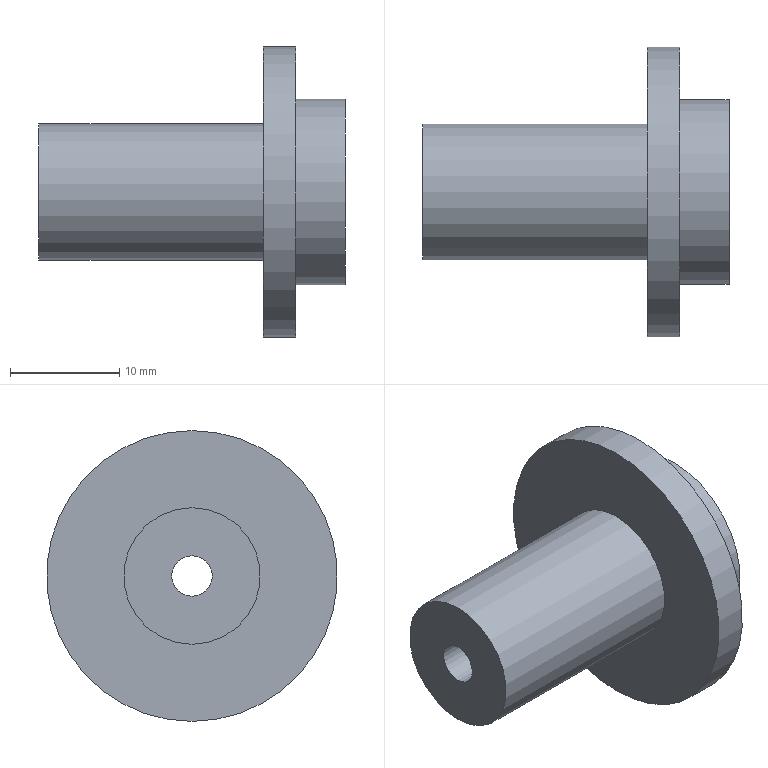Component | NX | FLOW_SEAT | 1 solid | 8 faces | box 28 x 26.6 x 26.6 mm | volume 4903 mm3 | cylinder 4 | plane 4 | commonest cylinder face diameters 12.5 x1 26.6 x1 17 x1 3.7 x1
STEP:
#1=CARTESIAN_POINT('',(0.,0.,0.));
#2=DIRECTION('',(0.,0.,1.));
#3=DIRECTION('',(1.,0.,0.));
#4=AXIS2_PLACEMENT_3D('',#1,#2,#3);
#5=CARTESIAN_POINT('',(-8.,-0.,13.75));
#6=VERTEX_POINT('',#5);
#7=CARTESIAN_POINT('',(-8.,-0.,20.));
#8=DIRECTION('',(1.,0.,0.));
#9=DIRECTION('',(0.,0.,-1.));
#10=AXIS2_PLACEMENT_3D('',#7,#8,#9);
#11=CIRCLE('',#10,6.25);
#12=CARTESIAN_POINT('',(-8.,-0.,20.));
#13=DIRECTION('',(-1.,0.,0.));
#14=DIRECTION('',(0.,0.,1.));
#15=AXIS2_PLACEMENT_3D('',#12,#13,#14);
#16=CYLINDRICAL_SURFACE('',#15,6.25);
#17=CARTESIAN_POINT('',(9.425,0.));
#18=DIRECTION('',(-1.,0.));
#19=VECTOR('',#18,1.);
#20=LINE('',#17,#19);
#21=(GEOMETRIC_REPRESENTATION_CONTEXT(2)PARAMETRIC_REPRESENTATION_CONTEXT()REPRESENTATION_CONTEXT('',''));
#22=DEFINITIONAL_REPRESENTATION('',(#20),#21);
#23=PCURVE('',#16,#22);
#24=CARTESIAN_POINT('',(-8.,-0.,20.));
#25=DIRECTION('',(1.,0.,0.));
#26=DIRECTION('',(0.,0.,-1.));
#27=AXIS2_PLACEMENT_3D('',#24,#25,#26);
#28=PLANE('',#27);
#29=CARTESIAN_POINT('',(0.,0.));
#30=DIRECTION('',(1.,0.));
#31=AXIS2_PLACEMENT_2D('',#29,#30);
#32=CIRCLE('',#31,6.25);
#33=(GEOMETRIC_REPRESENTATION_CONTEXT(2)PARAMETRIC_REPRESENTATION_CONTEXT()REPRESENTATION_CONTEXT('',''));
#34=DEFINITIONAL_REPRESENTATION('',(#32),#33);
#35=PCURVE('',#28,#34);
#36=SURFACE_CURVE('',#11,(#23,#35),.PCURVE_S1.);
#37=EDGE_CURVE('',#6,#6,#36,.T.);
#38=ORIENTED_EDGE('',*,*,#37,.F.);
#39=CARTESIAN_POINT('',(-28.5,-0.,13.75));
#40=VERTEX_POINT('',#39);
#41=CARTESIAN_POINT('',(-8.,-0.,13.75));
#42=CARTESIAN_POINT('',(-28.5,-0.,13.75));
#43=B_SPLINE_CURVE_WITH_KNOTS('',1,(#41,#42),.UNSPECIFIED.,.F.,.F.,(2,2),(0.,20.5),.PIECEWISE_BEZIER_KNOTS.);
#44=CARTESIAN_POINT('',(9.425,0.));
#45=DIRECTION('',(0.,1.));
#46=VECTOR('',#45,1.);
#47=LINE('',#44,#46);
#48=(GEOMETRIC_REPRESENTATION_CONTEXT(2)PARAMETRIC_REPRESENTATION_CONTEXT()REPRESENTATION_CONTEXT('',''));
#49=DEFINITIONAL_REPRESENTATION('',(#47),#48);
#50=PCURVE('',#16,#49);
#51=CARTESIAN_POINT('',(3.142,0.));
#52=DIRECTION('',(0.,1.));
#53=VECTOR('',#52,1.);
#54=LINE('',#51,#53);
#55=(GEOMETRIC_REPRESENTATION_CONTEXT(2)PARAMETRIC_REPRESENTATION_CONTEXT()REPRESENTATION_CONTEXT('',''));
#56=DEFINITIONAL_REPRESENTATION('',(#54),#55);
#57=PCURVE('',#16,#56);
#58=SEAM_CURVE('',#43,(#50,#57),.PCURVE_S1.);
#59=EDGE_CURVE('',#6,#40,#58,.T.);
#60=ORIENTED_EDGE('',*,*,#59,.T.);
#61=CARTESIAN_POINT('',(-28.5,-0.,20.));
#62=DIRECTION('',(1.,0.,0.));
#63=DIRECTION('',(0.,0.,-1.));
#64=AXIS2_PLACEMENT_3D('',#61,#62,#63);
#65=CIRCLE('',#64,6.25);
#66=CARTESIAN_POINT('',(9.425,20.5));
#67=DIRECTION('',(-1.,0.));
#68=VECTOR('',#67,1.);
#69=LINE('',#66,#68);
#70=(GEOMETRIC_REPRESENTATION_CONTEXT(2)PARAMETRIC_REPRESENTATION_CONTEXT()REPRESENTATION_CONTEXT('',''));
#71=DEFINITIONAL_REPRESENTATION('',(#69),#70);
#72=PCURVE('',#16,#71);
#73=CARTESIAN_POINT('',(-28.5,-0.,20.));
#74=DIRECTION('',(1.,0.,0.));
#75=DIRECTION('',(0.,0.,-1.));
#76=AXIS2_PLACEMENT_3D('',#73,#74,#75);
#77=PLANE('',#76);
#78=CARTESIAN_POINT('',(0.,0.));
#79=DIRECTION('',(1.,0.));
#80=AXIS2_PLACEMENT_2D('',#78,#79);
#81=CIRCLE('',#80,6.25);
#82=(GEOMETRIC_REPRESENTATION_CONTEXT(2)PARAMETRIC_REPRESENTATION_CONTEXT()REPRESENTATION_CONTEXT('',''));
#83=DEFINITIONAL_REPRESENTATION('',(#81),#82);
#84=PCURVE('',#77,#83);
#85=SURFACE_CURVE('',#65,(#72,#84),.PCURVE_S1.);
#86=EDGE_CURVE('',#40,#40,#85,.T.);
#87=ORIENTED_EDGE('',*,*,#86,.T.);
#88=ORIENTED_EDGE('',*,*,#59,.F.);
#89=EDGE_LOOP('',(#38,#60,#87,#88));
#90=FACE_BOUND('',#89,.T.);
#91=ADVANCED_FACE('',(#90),#16,.T.);
#92=CARTESIAN_POINT('',(-28.5,-0.,18.15));
#93=VERTEX_POINT('',#92);
#94=CARTESIAN_POINT('',(-28.5,-0.,21.85));
#95=VERTEX_POINT('',#94);
#96=CARTESIAN_POINT('',(-28.5,-0.,20.));
#97=DIRECTION('',(1.,0.,0.));
#98=DIRECTION('',(0.,0.,-1.));
#99=AXIS2_PLACEMENT_3D('',#96,#97,#98);
#100=CIRCLE('',#99,1.85);
#101=CARTESIAN_POINT('',(0.,0.));
#102=DIRECTION('',(1.,0.));
#103=AXIS2_PLACEMENT_2D('',#101,#102);
#104=CIRCLE('',#103,1.85);
#105=(GEOMETRIC_REPRESENTATION_CONTEXT(2)PARAMETRIC_REPRESENTATION_CONTEXT()REPRESENTATION_CONTEXT('',''));
#106=DEFINITIONAL_REPRESENTATION('',(#104),#105);
#107=PCURVE('',#77,#106);
#108=CARTESIAN_POINT('',(-0.5,-0.,20.));
#109=DIRECTION('',(-1.,0.,0.));
#110=DIRECTION('',(0.,0.,1.));
#111=AXIS2_PLACEMENT_3D('',#108,#109,#110);
#112=CYLINDRICAL_SURFACE('',#111,1.85);
#113=CARTESIAN_POINT('',(3.142,28.));
#114=DIRECTION('',(-1.,0.));
#115=VECTOR('',#114,1.);
#116=LINE('',#113,#115);
#117=(GEOMETRIC_REPRESENTATION_CONTEXT(2)PARAMETRIC_REPRESENTATION_CONTEXT()REPRESENTATION_CONTEXT('',''));
#118=DEFINITIONAL_REPRESENTATION('',(#116),#117);
#119=PCURVE('',#112,#118);
#120=SURFACE_CURVE('',#100,(#107,#119),.PCURVE_S1.);
#121=EDGE_CURVE('',#93,#95,#120,.T.);
#122=ORIENTED_EDGE('',*,*,#121,.T.);
#123=CARTESIAN_POINT('',(-28.5,-0.,20.));
#124=DIRECTION('',(1.,0.,0.));
#125=DIRECTION('',(0.,0.,-1.));
#126=AXIS2_PLACEMENT_3D('',#123,#124,#125);
#127=CIRCLE('',#126,1.85);
#128=CARTESIAN_POINT('',(0.,0.));
#129=DIRECTION('',(1.,0.));
#130=AXIS2_PLACEMENT_2D('',#128,#129);
#131=CIRCLE('',#130,1.85);
#132=(GEOMETRIC_REPRESENTATION_CONTEXT(2)PARAMETRIC_REPRESENTATION_CONTEXT()REPRESENTATION_CONTEXT('',''));
#133=DEFINITIONAL_REPRESENTATION('',(#131),#132);
#134=PCURVE('',#77,#133);
#135=CARTESIAN_POINT('',(9.425,28.));
#136=DIRECTION('',(-1.,0.));
#137=VECTOR('',#136,1.);
#138=LINE('',#135,#137);
#139=(GEOMETRIC_REPRESENTATION_CONTEXT(2)PARAMETRIC_REPRESENTATION_CONTEXT()REPRESENTATION_CONTEXT('',''));
#140=DEFINITIONAL_REPRESENTATION('',(#138),#139);
#141=PCURVE('',#112,#140);
#142=SURFACE_CURVE('',#127,(#134,#141),.PCURVE_S1.);
#143=EDGE_CURVE('',#95,#93,#142,.T.);
#144=ORIENTED_EDGE('',*,*,#143,.T.);
#145=EDGE_LOOP('',(#122,#144));
#146=FACE_BOUND('',#145,.T.);
#147=ORIENTED_EDGE('',*,*,#86,.F.);
#148=EDGE_LOOP('',(#147));
#149=FACE_BOUND('',#148,.T.);
#150=ADVANCED_FACE('',(#146,#149),#77,.F.);
#151=CARTESIAN_POINT('',(-5.,-0.,6.7));
#152=VERTEX_POINT('',#151);
#153=CARTESIAN_POINT('',(-5.,-0.,20.));
#154=DIRECTION('',(1.,0.,0.));
#155=DIRECTION('',(0.,0.,-1.));
#156=AXIS2_PLACEMENT_3D('',#153,#154,#155);
#157=CIRCLE('',#156,13.3);
#158=CARTESIAN_POINT('',(-5.,-0.,20.));
#159=DIRECTION('',(-1.,0.,0.));
#160=DIRECTION('',(0.,0.,1.));
#161=AXIS2_PLACEMENT_3D('',#158,#159,#160);
#162=CYLINDRICAL_SURFACE('',#161,13.3);
#163=CARTESIAN_POINT('',(9.425,0.));
#164=DIRECTION('',(-1.,0.));
#165=VECTOR('',#164,1.);
#166=LINE('',#163,#165);
#167=(GEOMETRIC_REPRESENTATION_CONTEXT(2)PARAMETRIC_REPRESENTATION_CONTEXT()REPRESENTATION_CONTEXT('',''));
#168=DEFINITIONAL_REPRESENTATION('',(#166),#167);
#169=PCURVE('',#162,#168);
#170=CARTESIAN_POINT('',(-5.,-0.,20.));
#171=DIRECTION('',(1.,0.,0.));
#172=DIRECTION('',(0.,0.,-1.));
#173=AXIS2_PLACEMENT_3D('',#170,#171,#172);
#174=PLANE('',#173);
#175=CARTESIAN_POINT('',(0.,0.));
#176=DIRECTION('',(1.,0.));
#177=AXIS2_PLACEMENT_2D('',#175,#176);
#178=CIRCLE('',#177,13.3);
#179=(GEOMETRIC_REPRESENTATION_CONTEXT(2)PARAMETRIC_REPRESENTATION_CONTEXT()REPRESENTATION_CONTEXT('',''));
#180=DEFINITIONAL_REPRESENTATION('',(#178),#179);
#181=PCURVE('',#174,#180);
#182=SURFACE_CURVE('',#157,(#169,#181),.PCURVE_S1.);
#183=EDGE_CURVE('',#152,#152,#182,.T.);
#184=ORIENTED_EDGE('',*,*,#183,.F.);
#185=CARTESIAN_POINT('',(-8.,-0.,6.7));
#186=VERTEX_POINT('',#185);
#187=CARTESIAN_POINT('',(-5.,-0.,6.7));
#188=CARTESIAN_POINT('',(-8.,-0.,6.7));
#189=B_SPLINE_CURVE_WITH_KNOTS('',1,(#187,#188),.UNSPECIFIED.,.F.,.F.,(2,2),(0.,3.),.PIECEWISE_BEZIER_KNOTS.);
#190=CARTESIAN_POINT('',(9.425,0.));
#191=DIRECTION('',(0.,1.));
#192=VECTOR('',#191,1.);
#193=LINE('',#190,#192);
#194=(GEOMETRIC_REPRESENTATION_CONTEXT(2)PARAMETRIC_REPRESENTATION_CONTEXT()REPRESENTATION_CONTEXT('',''));
#195=DEFINITIONAL_REPRESENTATION('',(#193),#194);
#196=PCURVE('',#162,#195);
#197=CARTESIAN_POINT('',(3.142,0.));
#198=DIRECTION('',(0.,1.));
#199=VECTOR('',#198,1.);
#200=LINE('',#197,#199);
#201=(GEOMETRIC_REPRESENTATION_CONTEXT(2)PARAMETRIC_REPRESENTATION_CONTEXT()REPRESENTATION_CONTEXT('',''));
#202=DEFINITIONAL_REPRESENTATION('',(#200),#201);
#203=PCURVE('',#162,#202);
#204=SEAM_CURVE('',#189,(#196,#203),.PCURVE_S1.);
#205=EDGE_CURVE('',#152,#186,#204,.T.);
#206=ORIENTED_EDGE('',*,*,#205,.T.);
#207=CARTESIAN_POINT('',(-8.,-0.,20.));
#208=DIRECTION('',(1.,0.,0.));
#209=DIRECTION('',(0.,0.,-1.));
#210=AXIS2_PLACEMENT_3D('',#207,#208,#209);
#211=CIRCLE('',#210,13.3);
#212=CARTESIAN_POINT('',(9.425,3.));
#213=DIRECTION('',(-1.,0.));
#214=VECTOR('',#213,1.);
#215=LINE('',#212,#214);
#216=(GEOMETRIC_REPRESENTATION_CONTEXT(2)PARAMETRIC_REPRESENTATION_CONTEXT()REPRESENTATION_CONTEXT('',''));
#217=DEFINITIONAL_REPRESENTATION('',(#215),#216);
#218=PCURVE('',#162,#217);
#219=CARTESIAN_POINT('',(0.,0.));
#220=DIRECTION('',(1.,0.));
#221=AXIS2_PLACEMENT_2D('',#219,#220);
#222=CIRCLE('',#221,13.3);
#223=(GEOMETRIC_REPRESENTATION_CONTEXT(2)PARAMETRIC_REPRESENTATION_CONTEXT()REPRESENTATION_CONTEXT('',''));
#224=DEFINITIONAL_REPRESENTATION('',(#222),#223);
#225=PCURVE('',#28,#224);
#226=SURFACE_CURVE('',#211,(#218,#225),.PCURVE_S1.);
#227=EDGE_CURVE('',#186,#186,#226,.T.);
#228=ORIENTED_EDGE('',*,*,#227,.T.);
#229=ORIENTED_EDGE('',*,*,#205,.F.);
#230=EDGE_LOOP('',(#184,#206,#228,#229));
#231=FACE_BOUND('',#230,.T.);
#232=ADVANCED_FACE('',(#231),#162,.T.);
#233=CARTESIAN_POINT('',(-5.,-0.,11.5));
#234=VERTEX_POINT('',#233);
#235=CARTESIAN_POINT('',(-5.,-0.,20.));
#236=DIRECTION('',(1.,0.,0.));
#237=DIRECTION('',(0.,0.,-1.));
#238=AXIS2_PLACEMENT_3D('',#235,#236,#237);
#239=CIRCLE('',#238,8.5);
#240=CARTESIAN_POINT('',(0.,0.));
#241=DIRECTION('',(1.,0.));
#242=AXIS2_PLACEMENT_2D('',#240,#241);
#243=CIRCLE('',#242,8.5);
#244=(GEOMETRIC_REPRESENTATION_CONTEXT(2)PARAMETRIC_REPRESENTATION_CONTEXT()REPRESENTATION_CONTEXT('',''));
#245=DEFINITIONAL_REPRESENTATION('',(#243),#244);
#246=PCURVE('',#174,#245);
#247=CARTESIAN_POINT('',(-0.5,-0.,20.));
#248=DIRECTION('',(-1.,0.,0.));
#249=DIRECTION('',(0.,0.,1.));
#250=AXIS2_PLACEMENT_3D('',#247,#248,#249);
#251=CYLINDRICAL_SURFACE('',#250,8.5);
#252=CARTESIAN_POINT('',(9.425,4.5));
#253=DIRECTION('',(-1.,0.));
#254=VECTOR('',#253,1.);
#255=LINE('',#252,#254);
#256=(GEOMETRIC_REPRESENTATION_CONTEXT(2)PARAMETRIC_REPRESENTATION_CONTEXT()REPRESENTATION_CONTEXT('',''));
#257=DEFINITIONAL_REPRESENTATION('',(#255),#256);
#258=PCURVE('',#251,#257);
#259=SURFACE_CURVE('',#239,(#246,#258),.PCURVE_S1.);
#260=EDGE_CURVE('',#234,#234,#259,.T.);
#261=ORIENTED_EDGE('',*,*,#260,.F.);
#262=EDGE_LOOP('',(#261));
#263=FACE_BOUND('',#262,.T.);
#264=ORIENTED_EDGE('',*,*,#183,.T.);
#265=EDGE_LOOP('',(#264));
#266=FACE_BOUND('',#265,.T.);
#267=ADVANCED_FACE('',(#263,#266),#174,.T.);
#268=ORIENTED_EDGE('',*,*,#37,.T.);
#269=EDGE_LOOP('',(#268));
#270=FACE_BOUND('',#269,.T.);
#271=ORIENTED_EDGE('',*,*,#227,.F.);
#272=EDGE_LOOP('',(#271));
#273=FACE_BOUND('',#272,.T.);
#274=ADVANCED_FACE('',(#270,#273),#28,.F.);
#275=CARTESIAN_POINT('',(-0.5,-0.,11.5));
#276=VERTEX_POINT('',#275);
#277=CARTESIAN_POINT('',(-0.5,-0.,20.));
#278=DIRECTION('',(1.,0.,0.));
#279=DIRECTION('',(0.,0.,-1.));
#280=AXIS2_PLACEMENT_3D('',#277,#278,#279);
#281=CIRCLE('',#280,8.5);
#282=CARTESIAN_POINT('',(9.425,0.));
#283=DIRECTION('',(-1.,0.));
#284=VECTOR('',#283,1.);
#285=LINE('',#282,#284);
#286=(GEOMETRIC_REPRESENTATION_CONTEXT(2)PARAMETRIC_REPRESENTATION_CONTEXT()REPRESENTATION_CONTEXT('',''));
#287=DEFINITIONAL_REPRESENTATION('',(#285),#286);
#288=PCURVE('',#251,#287);
#289=CARTESIAN_POINT('',(-0.5,-0.,20.));
#290=DIRECTION('',(1.,0.,0.));
#291=DIRECTION('',(0.,0.,-1.));
#292=AXIS2_PLACEMENT_3D('',#289,#290,#291);
#293=PLANE('',#292);
#294=CARTESIAN_POINT('',(0.,0.));
#295=DIRECTION('',(1.,0.));
#296=AXIS2_PLACEMENT_2D('',#294,#295);
#297=CIRCLE('',#296,8.5);
#298=(GEOMETRIC_REPRESENTATION_CONTEXT(2)PARAMETRIC_REPRESENTATION_CONTEXT()REPRESENTATION_CONTEXT('',''));
#299=DEFINITIONAL_REPRESENTATION('',(#297),#298);
#300=PCURVE('',#293,#299);
#301=SURFACE_CURVE('',#281,(#288,#300),.PCURVE_S1.);
#302=EDGE_CURVE('',#276,#276,#301,.T.);
#303=ORIENTED_EDGE('',*,*,#302,.F.);
#304=CARTESIAN_POINT('',(-0.5,-0.,11.5));
#305=CARTESIAN_POINT('',(-5.,-0.,11.5));
#306=B_SPLINE_CURVE_WITH_KNOTS('',1,(#304,#305),.UNSPECIFIED.,.F.,.F.,(2,2),(0.,4.5),.PIECEWISE_BEZIER_KNOTS.);
#307=CARTESIAN_POINT('',(9.425,0.));
#308=DIRECTION('',(0.,1.));
#309=VECTOR('',#308,1.);
#310=LINE('',#307,#309);
#311=(GEOMETRIC_REPRESENTATION_CONTEXT(2)PARAMETRIC_REPRESENTATION_CONTEXT()REPRESENTATION_CONTEXT('',''));
#312=DEFINITIONAL_REPRESENTATION('',(#310),#311);
#313=PCURVE('',#251,#312);
#314=CARTESIAN_POINT('',(3.142,0.));
#315=DIRECTION('',(0.,1.));
#316=VECTOR('',#315,1.);
#317=LINE('',#314,#316);
#318=(GEOMETRIC_REPRESENTATION_CONTEXT(2)PARAMETRIC_REPRESENTATION_CONTEXT()REPRESENTATION_CONTEXT('',''));
#319=DEFINITIONAL_REPRESENTATION('',(#317),#318);
#320=PCURVE('',#251,#319);
#321=SEAM_CURVE('',#306,(#313,#320),.PCURVE_S1.);
#322=EDGE_CURVE('',#276,#234,#321,.T.);
#323=ORIENTED_EDGE('',*,*,#322,.T.);
#324=ORIENTED_EDGE('',*,*,#260,.T.);
#325=ORIENTED_EDGE('',*,*,#322,.F.);
#326=EDGE_LOOP('',(#303,#323,#324,#325));
#327=FACE_BOUND('',#326,.T.);
#328=ADVANCED_FACE('',(#327),#251,.T.);
#329=CARTESIAN_POINT('',(-0.5,-0.,21.85));
#330=VERTEX_POINT('',#329);
#331=CARTESIAN_POINT('',(-0.5,-0.,20.));
#332=DIRECTION('',(-1.,0.,0.));
#333=DIRECTION('',(0.,0.,1.));
#334=AXIS2_PLACEMENT_3D('',#331,#332,#333);
#335=CIRCLE('',#334,1.85);
#336=CARTESIAN_POINT('',(-1.85,0.));
#337=CARTESIAN_POINT('',(-1.85,3.204));
#338=CARTESIAN_POINT('',(0.925,1.602));
#339=CARTESIAN_POINT('',(3.7,0.));
#340=CARTESIAN_POINT('',(0.925,-1.602));
#341=CARTESIAN_POINT('',(-1.85,-3.204));
#342=CARTESIAN_POINT('',(-1.85,0.));
#343=(BOUNDED_CURVE()B_SPLINE_CURVE(2,(#336,#337,#338,#339,#340,#341,#342),.UNSPECIFIED.,.T.,.F.)B_SPLINE_CURVE_WITH_KNOTS((1,2,2,2,2,1),(-2.094,0.,2.094,4.189,6.283,8.378),.UNSPECIFIED.)CURVE()GEOMETRIC_REPRESENTATION_ITEM()RATIONAL_B_SPLINE_CURVE((1.,0.5,1.,0.5,1.,0.5,1.))REPRESENTATION_ITEM(''));
#344=(GEOMETRIC_REPRESENTATION_CONTEXT(2)PARAMETRIC_REPRESENTATION_CONTEXT()REPRESENTATION_CONTEXT('',''));
#345=DEFINITIONAL_REPRESENTATION('',(#343),#344);
#346=PCURVE('',#293,#345);
#347=CARTESIAN_POINT('',(0.,0.));
#348=DIRECTION('',(1.,0.));
#349=VECTOR('',#348,1.);
#350=LINE('',#347,#349);
#351=(GEOMETRIC_REPRESENTATION_CONTEXT(2)PARAMETRIC_REPRESENTATION_CONTEXT()REPRESENTATION_CONTEXT('',''));
#352=DEFINITIONAL_REPRESENTATION('',(#350),#351);
#353=PCURVE('',#112,#352);
#354=SURFACE_CURVE('',#335,(#346,#353),.PCURVE_S1.);
#355=EDGE_CURVE('',#330,#330,#354,.T.);
#356=ORIENTED_EDGE('',*,*,#355,.T.);
#357=EDGE_LOOP('',(#356));
#358=FACE_BOUND('',#357,.T.);
#359=ORIENTED_EDGE('',*,*,#302,.T.);
#360=EDGE_LOOP('',(#359));
#361=FACE_BOUND('',#360,.T.);
#362=ADVANCED_FACE('',(#358,#361),#293,.T.);
#363=ORIENTED_EDGE('',*,*,#355,.T.);
#364=CARTESIAN_POINT('',(-0.5,-0.,21.85));
#365=CARTESIAN_POINT('',(-28.5,-0.,21.85));
#366=B_SPLINE_CURVE_WITH_KNOTS('',1,(#364,#365),.UNSPECIFIED.,.F.,.F.,(2,2),(0.,28.),.PIECEWISE_BEZIER_KNOTS.);
#367=CARTESIAN_POINT('',(6.283,0.));
#368=DIRECTION('',(0.,1.));
#369=VECTOR('',#368,1.);
#370=LINE('',#367,#369);
#371=(GEOMETRIC_REPRESENTATION_CONTEXT(2)PARAMETRIC_REPRESENTATION_CONTEXT()REPRESENTATION_CONTEXT('',''));
#372=DEFINITIONAL_REPRESENTATION('',(#370),#371);
#373=PCURVE('',#112,#372);
#374=CARTESIAN_POINT('',(0.,0.));
#375=DIRECTION('',(0.,1.));
#376=VECTOR('',#375,1.);
#377=LINE('',#374,#376);
#378=(GEOMETRIC_REPRESENTATION_CONTEXT(2)PARAMETRIC_REPRESENTATION_CONTEXT()REPRESENTATION_CONTEXT('',''));
#379=DEFINITIONAL_REPRESENTATION('',(#377),#378);
#380=PCURVE('',#112,#379);
#381=SEAM_CURVE('',#366,(#373,#380),.PCURVE_S1.);
#382=EDGE_CURVE('',#330,#95,#381,.T.);
#383=ORIENTED_EDGE('',*,*,#382,.T.);
#384=ORIENTED_EDGE('',*,*,#143,.T.);
#385=ORIENTED_EDGE('',*,*,#121,.T.);
#386=ORIENTED_EDGE('',*,*,#382,.F.);
#387=EDGE_LOOP('',(#363,#383,#384,#385,#386));
#388=FACE_BOUND('',#387,.F.);
#389=ADVANCED_FACE('',(#388),#112,.F.);
#390=CLOSED_SHELL('',(#91,#150,#232,#267,#274,#328,#362,#389));
#391=MANIFOLD_SOLID_BREP('',#390);
#392=(LENGTH_UNIT()NAMED_UNIT(*)SI_UNIT(.MILLI.,.METRE.));
#393=UNCERTAINTY_MEASURE_WITH_UNIT(LENGTH_MEASURE(0.000005),#392,'','');
#394=(NAMED_UNIT(*)PLANE_ANGLE_UNIT()SI_UNIT($,.RADIAN.));
#395=(NAMED_UNIT(*)SI_UNIT($,.STERADIAN.)SOLID_ANGLE_UNIT());
#396=(GEOMETRIC_REPRESENTATION_CONTEXT(3)GLOBAL_UNCERTAINTY_ASSIGNED_CONTEXT((#393))GLOBAL_UNIT_ASSIGNED_CONTEXT((#392,#394,#395))REPRESENTATION_CONTEXT('',''));
#397=ADVANCED_BREP_SHAPE_REPRESENTATION('',(#4,#391),#396);